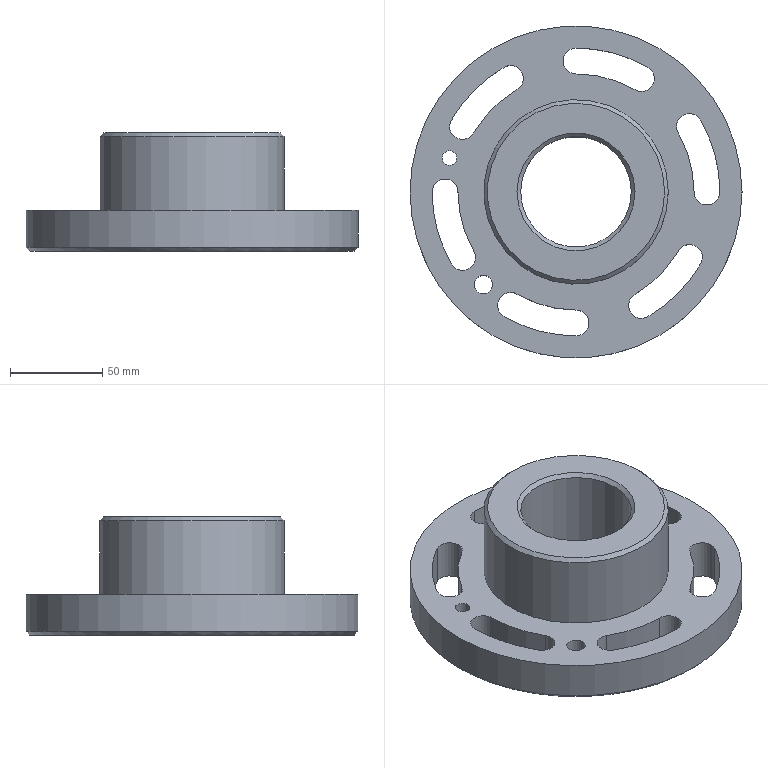CAM job | NX | mm | 3+2-indexed | 1 set-up | 10 operations | part box 180 x 180 x 64
set-up 1
1. Cavity Milling | Mill Mill5 D16 | CAVITY_MILL | path 296133.41 mm | 141.36 min
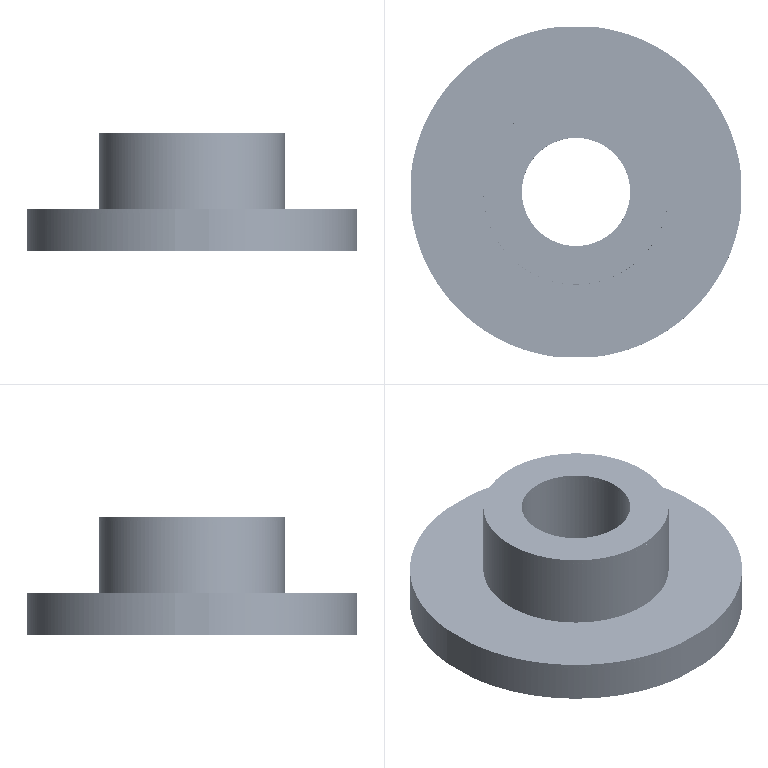2. Cavity Milling | Mill Mill5 D10 | CAVITY_MILL_1 | path 10776.742 mm | 5.524 min
3. Cavity Milling | Mill Mill5 D6 | CAVITY_MILL_2 | path 3496.597 mm | 0.7224 min
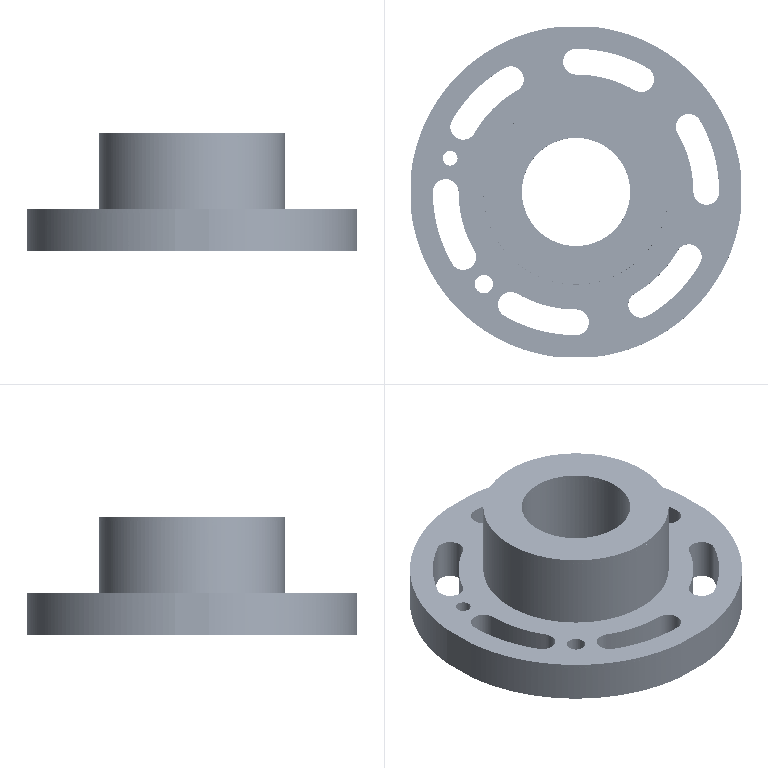4. Volume Based 2.5D Milling | Mill Mill5 D10 | FLOOR_WALL | path 6926.502 mm | 8.333 min
5. Planar Milling | Mill Mill5 D10 | PLANAR_PROFILE | path 450.783 mm | 0.4623 min
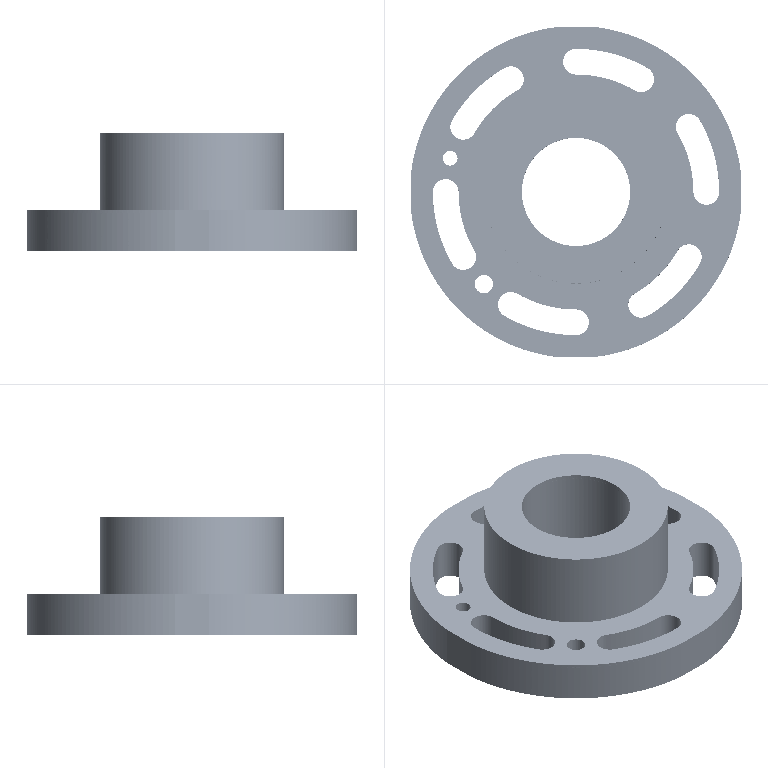6. Planar Milling | Mill Mill5 D10 | PLANAR_PROFILE_COPY | path 6059.405 mm | 4.649 min
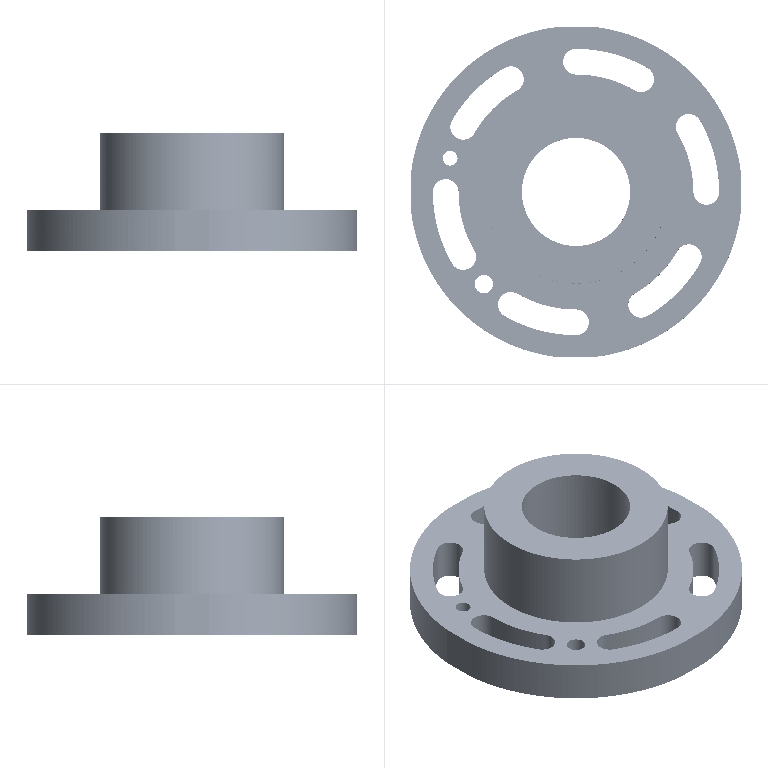7. Volume Based 2.5D Milling | Mill Mill5 D8DJ | FLOOR_WALL_1 | path 221.258 mm | 0.8616 min
8. Cavity Milling | Mill Mill5 D16 | CAVITY_MILL_COPY | path 4548.225 mm | 2.972 min
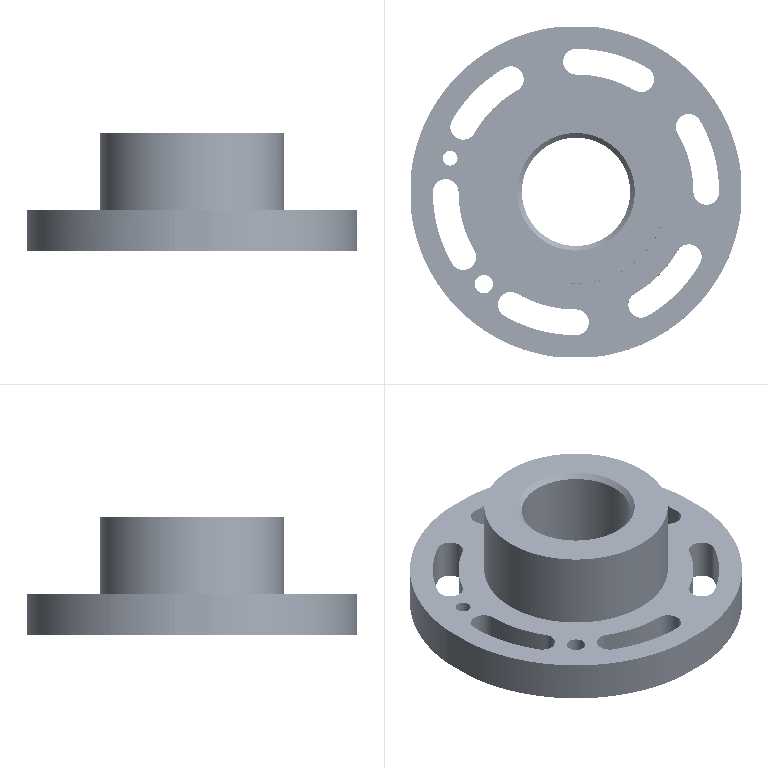9. Volume Based 2.5D Milling | Mill Mill5 D8DJ | FLOOR_WALL_1_COPY | path 215.258 mm | 0.861 min
10. Planar Milling | Mill Mill5 D8DJ | PLANAR_MILL | path 340.301 mm | 0.8292 min